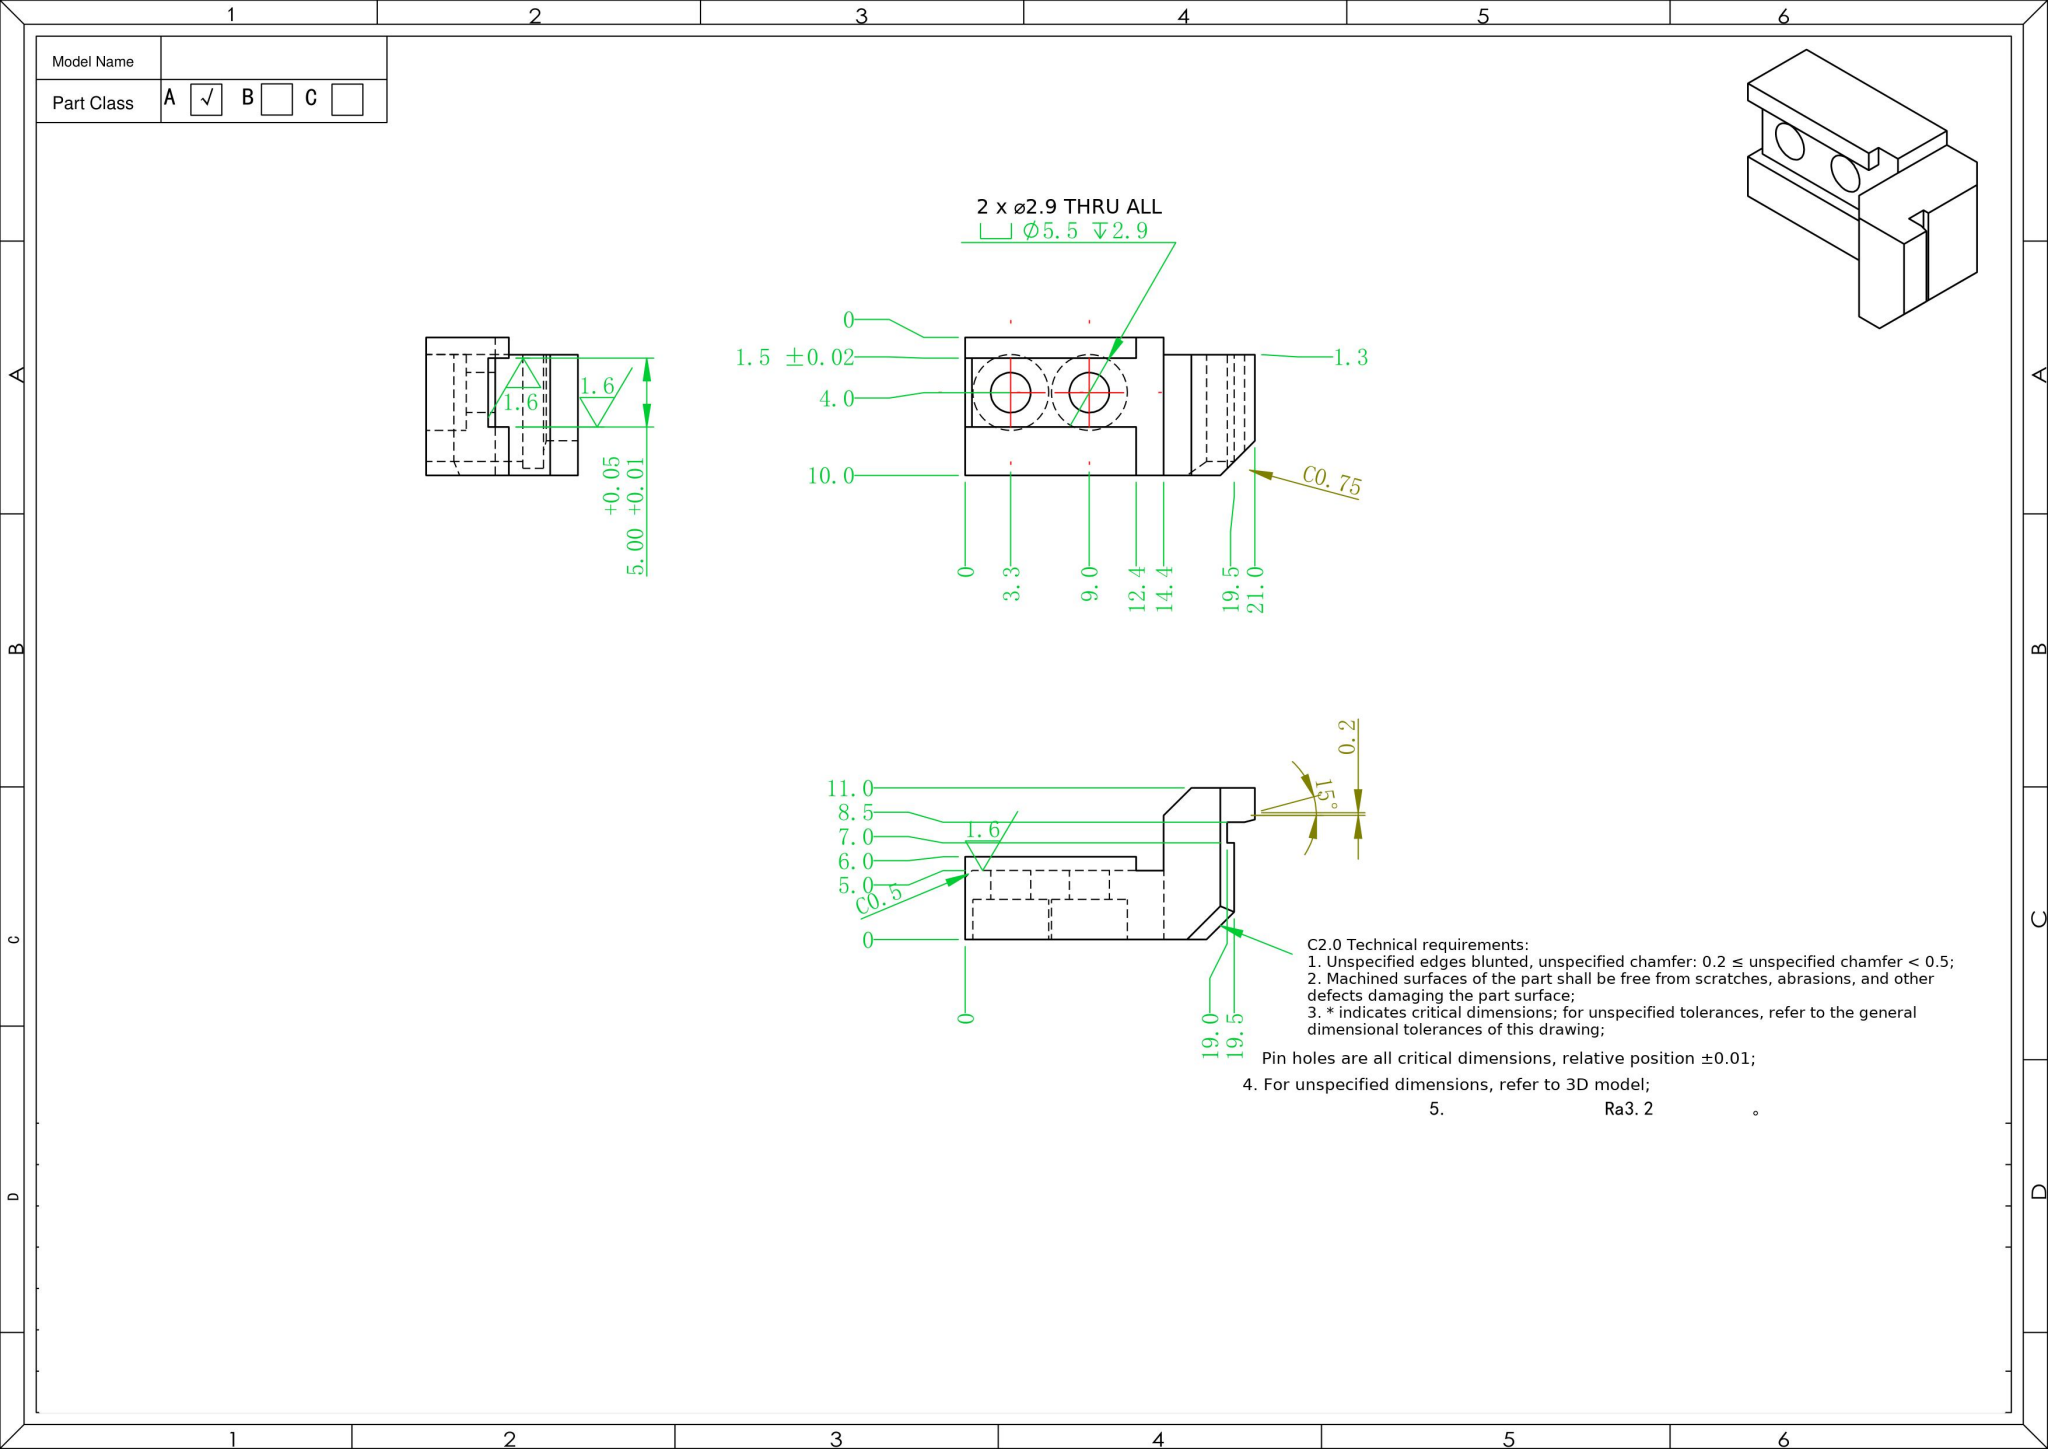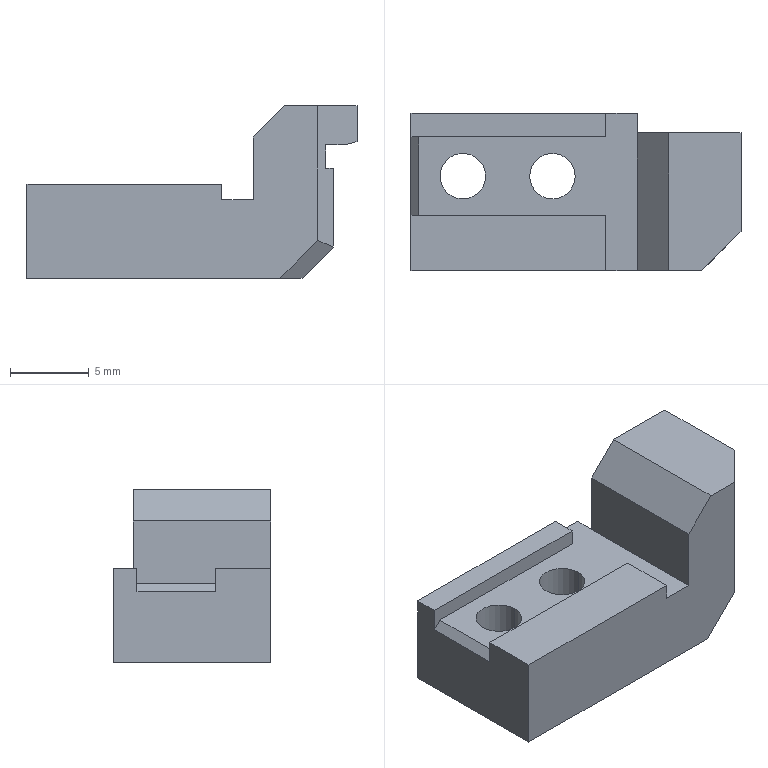Part | SolidWorks | mm | 1 solid | 36 faces | box 21 x 10 x 11 mm | volume 1086 mm3 | plane 28 | cylinder 8 | commonest cylinder face diameters 5.5 x4 2.9 x4